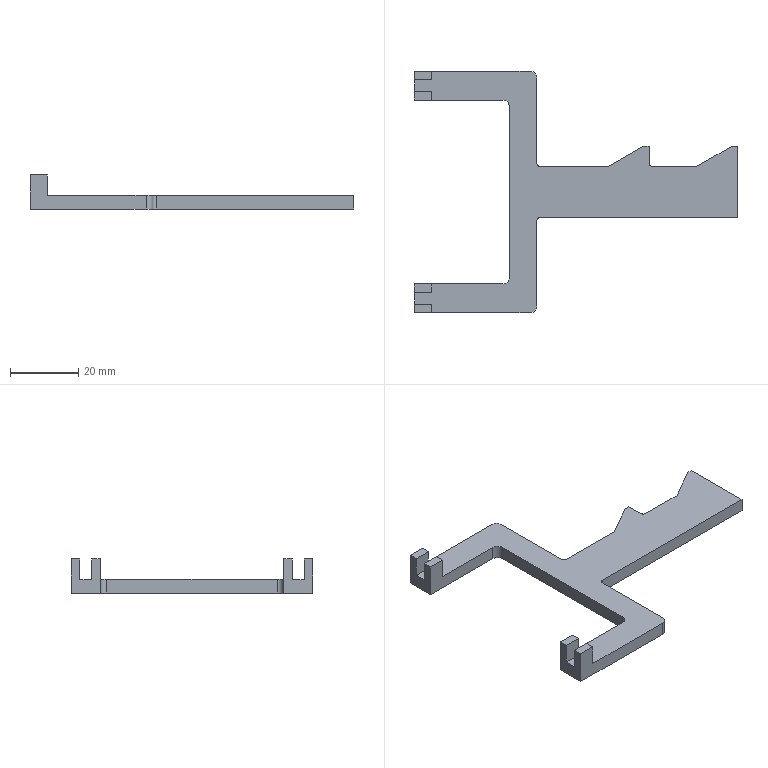Component | SolidWorks | ConnectingRod-1 | 1 solid | 39 faces | box 95 x 71 x 10 mm | volume 8345 mm3 | plane 32 | cylinder 7 | commonest cylinder face diameters 4 x4 2 x3
build123d program:
from build123d import *

# Parameters (mm, degrees)
SKETCH1_W             = 95
SKETCH1_H             = 71
EXTRUDE1_DEPTH        = 4
SKETCH2_W             = 28
SKETCH2_H             = 54
SKETCH2_W_2           = 59
SKETCH2_H_2           = 28
EXTRUDE2_DEPTH        = 5
SKETCH3_W             = 5
SKETCH3_H             = 8.5
EXTRUDE3_DEPTH        = 6
SKETCH4_W             = 6
SKETCH4_H             = 3.5
EXTRUDE4_DEPTH        = 98.264
EXTRUDE5_DEPTH        = 4
LINEAR_PATTERN1_COUNT = 2
LINEAR_PATTERN1_PITCH = 26
FILLET1_R             = 1
FILLET2_R             = 1
FILLET3_R             = 2


with BuildPart() as part:
    # Sketch1 → Extrude1 (new body)
    with BuildSketch(Plane.XY):
        Rectangle(SKETCH1_W, SKETCH1_H)
    extrude(amount=EXTRUDE1_DEPTH)

    # Sketch2 → Extrude2 (cut)
    with BuildSketch(Plane.XY.offset(4)):
        with Locations((-33.5, 0)):
            Rectangle(SKETCH2_W, SKETCH2_H)
        with Locations((18, -21.5)):
            Rectangle(SKETCH2_W_2, SKETCH2_H_2)
        with Locations((18, 21.5)):
            Rectangle(SKETCH2_W_2, SKETCH2_H_2)
    extrude(amount=-EXTRUDE2_DEPTH, mode=Mode.SUBTRACT)

    # Sketch3 → Extrude3 (add)
    with BuildSketch(Plane.XY.offset(4)):
        with Locations((-45, 31.25)):
            Rectangle(SKETCH3_W, SKETCH3_H)
        with Locations((-45, -31.25)):
            Rectangle(SKETCH3_W, SKETCH3_H)
    extrude(amount=EXTRUDE3_DEPTH)

    # Sketch4 → Extrude4 (cut, through all)
    with BuildSketch(Plane(origin=(-42.5, 0, 0), x_dir=(0, 0, -1), z_dir=(1, 0, 0))):
        with Locations((-7, 31.25)):
            Rectangle(SKETCH4_W, SKETCH4_H)
    extrude4 = extrude(amount=-EXTRUDE4_DEPTH, mode=Mode.SUBTRACT)

    # Mirror1: Extrude4 across plane
    add(extrude4.mirror(Plane.ZX), mode=Mode.SUBTRACT)

    # Sketch5 → Extrude5 (add)
    with BuildSketch(Plane.XY.offset(4)):
        Polygon((47.5, 7.5), (47.5, 13.5), (45.892, 13.5), (35.5, 7.5), align=None)
    extrude5 = extrude(amount=-EXTRUDE5_DEPTH)

    # Linear Pattern1: Extrude5 ×2
    with Locations(*[(-i * LINEAR_PATTERN1_PITCH, 0, 0) for i in range(1, LINEAR_PATTERN1_COUNT)]):
        add(extrude5)

    # Fillet1
    fillet1_edges = [part.edges().sort_by_distance(p)[0] for p in [
        (21.5, 7.5, 2),
    ]]
    fillet(fillet1_edges, radius=FILLET1_R)

    # Fillet2
    fillet2_edges = [part.edges().sort_by_distance(p)[0] for p in [
        (-11.5, 7.5, 2),
        (-11.5, -7.5, 2),
    ]]
    fillet(fillet2_edges, radius=FILLET2_R)

    # Fillet3
    fillet3_edges = [part.edges().sort_by_distance(p)[0] for p in [
        (-11.5, -35.5, 2),
        (-11.5, 35.5, 2),
        (-19.5, 27, 2),
        (-19.5, -27, 2),
    ]]
    fillet(fillet3_edges, radius=FILLET3_R)


solid = part.part

# Placed as in the assembly
solid = solid.moved(Location((-16.5, 0, 10), (0, 0, 0)))